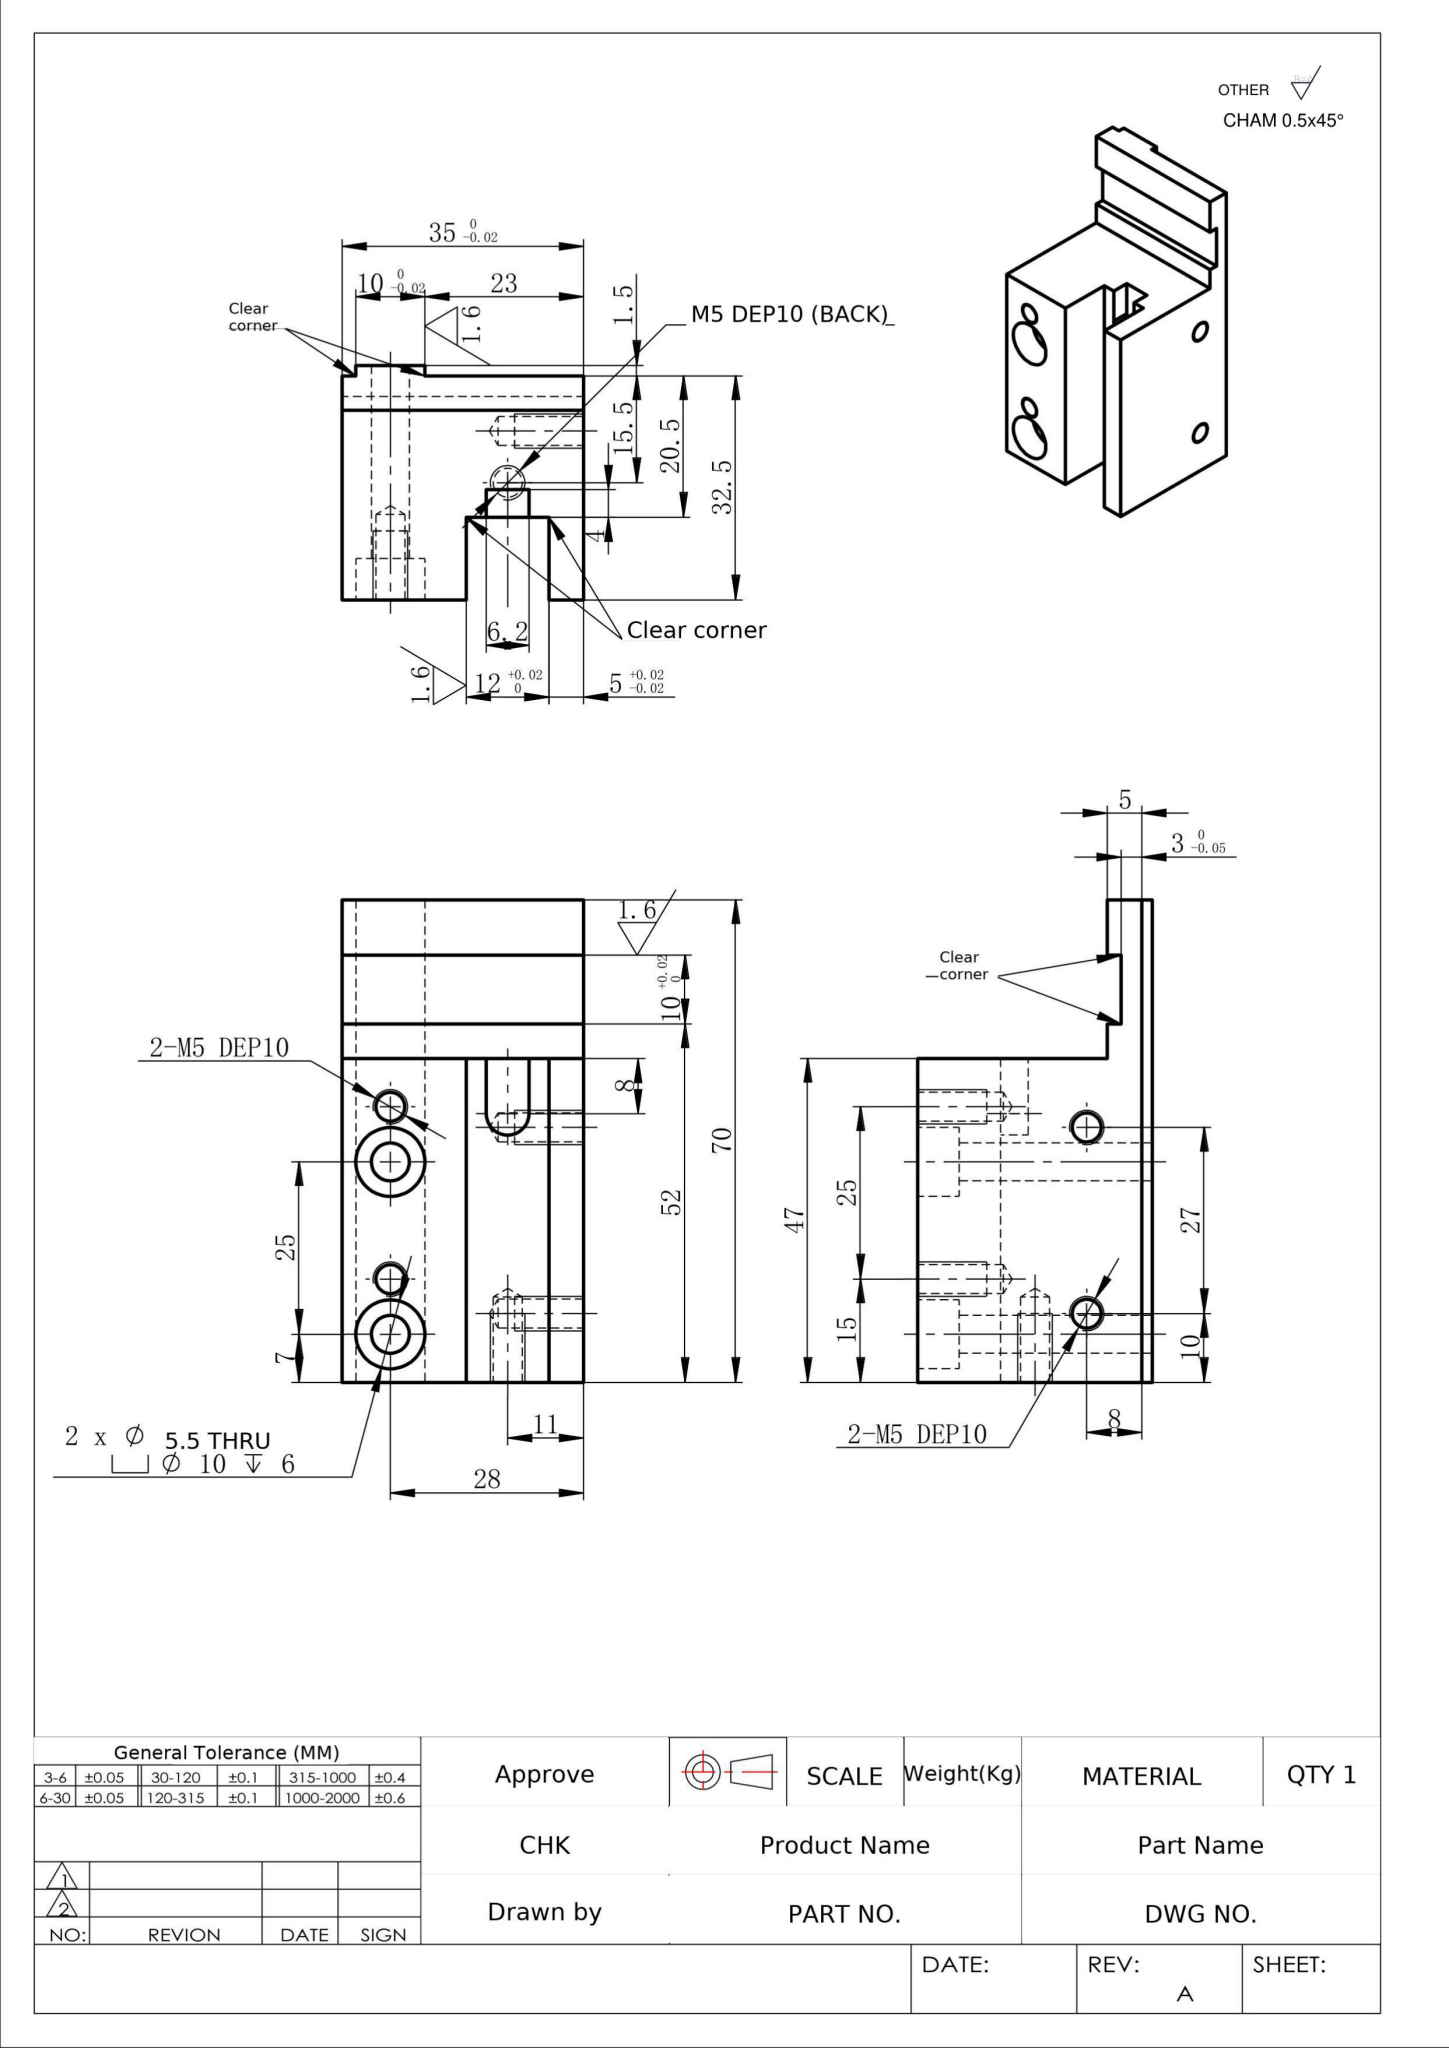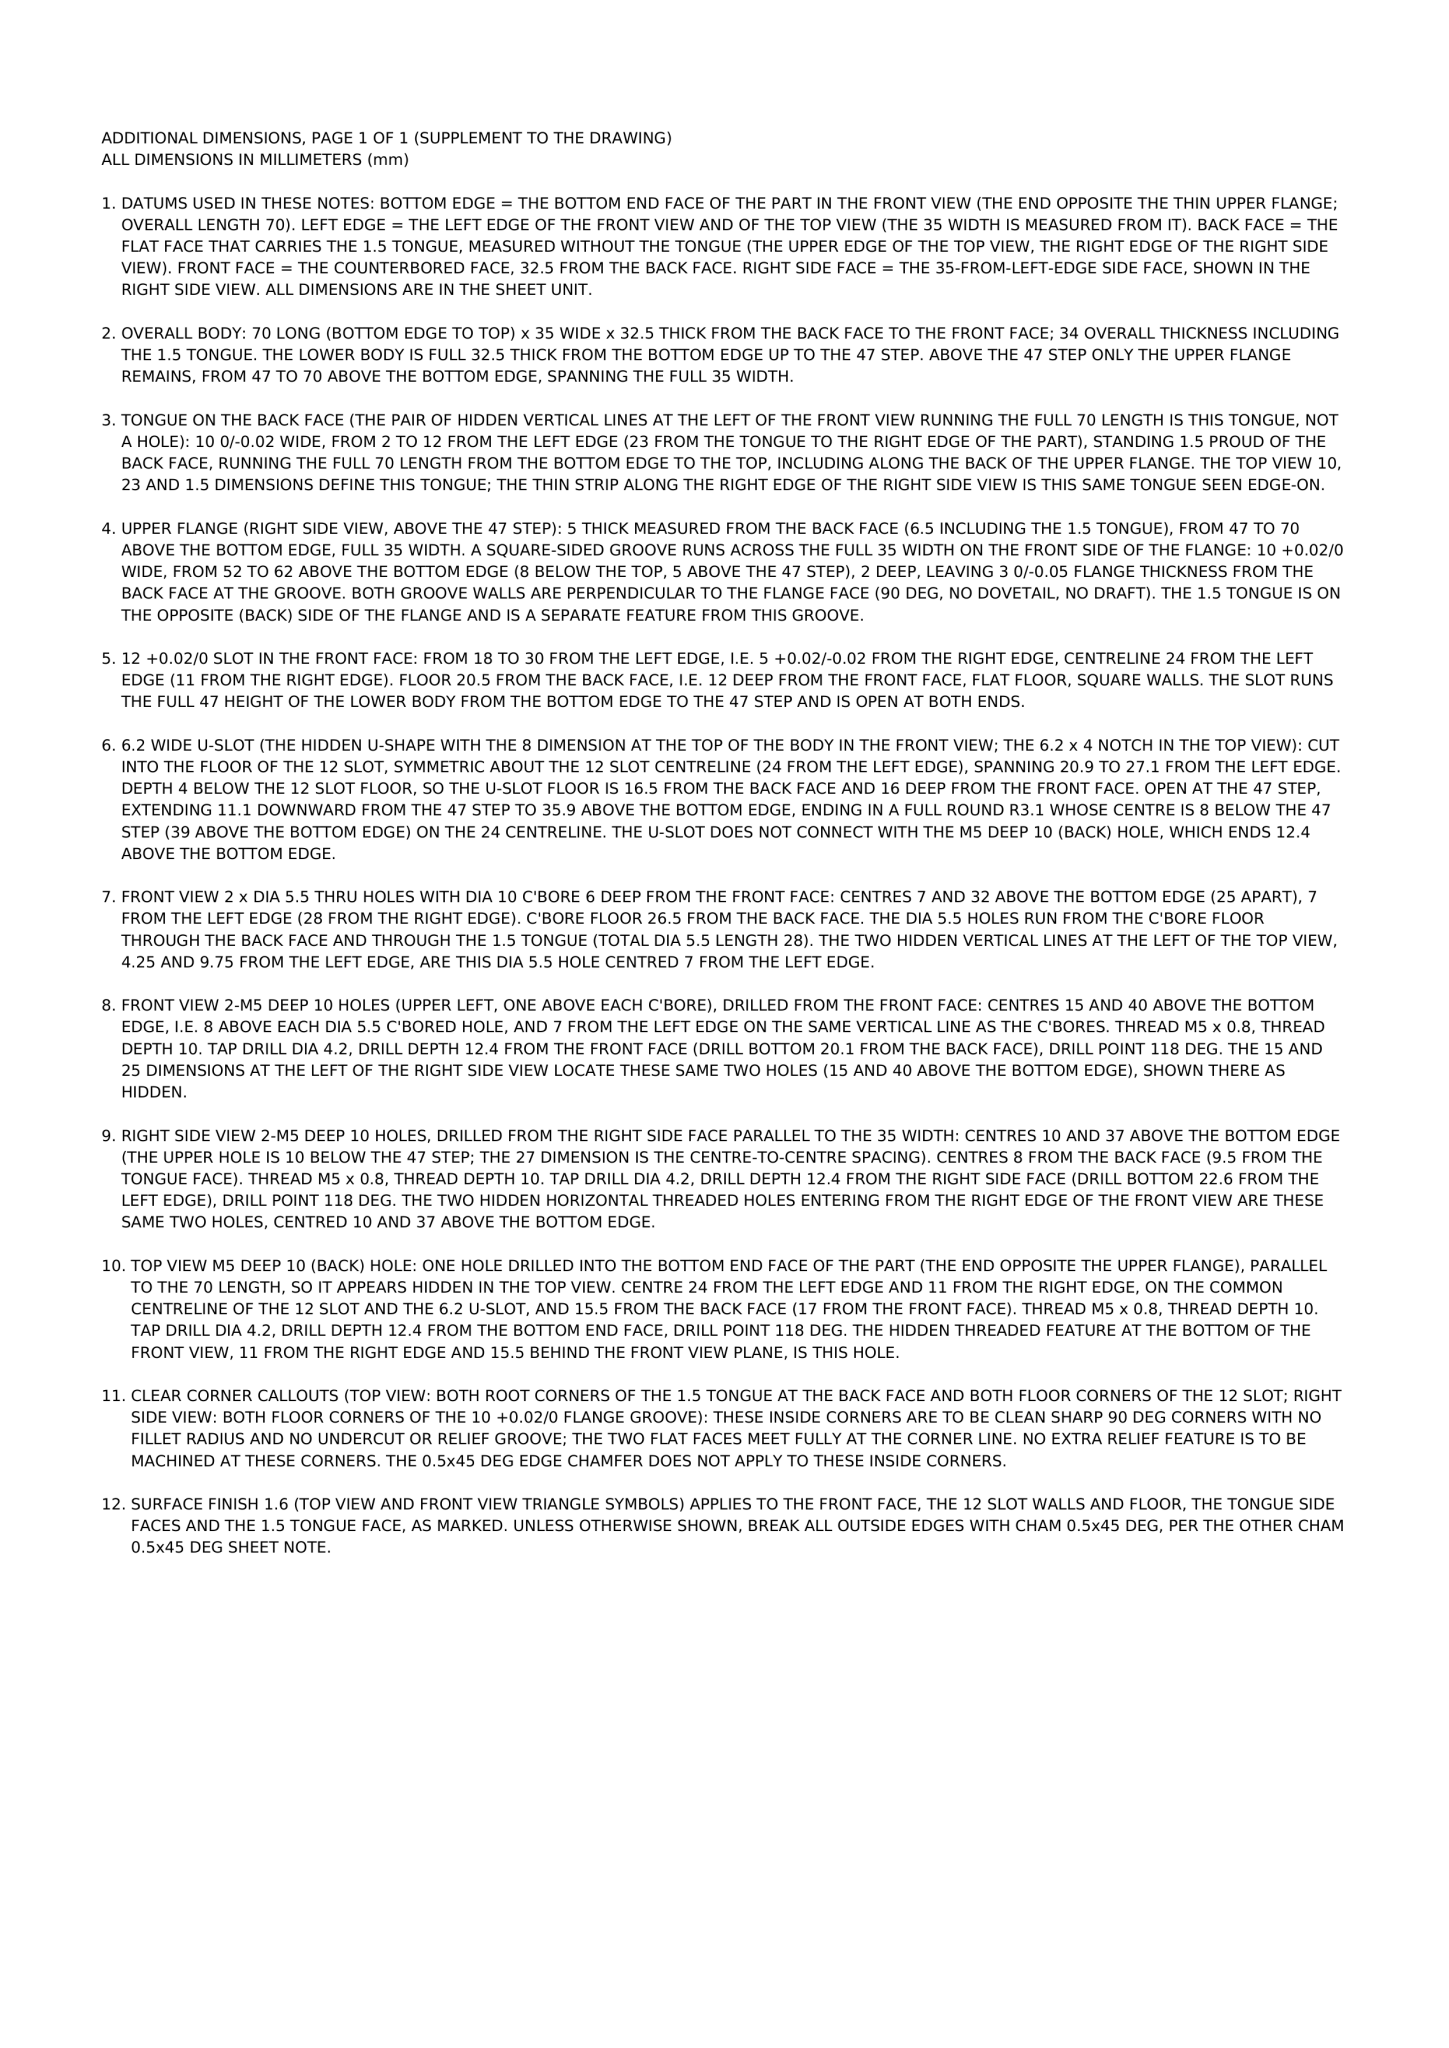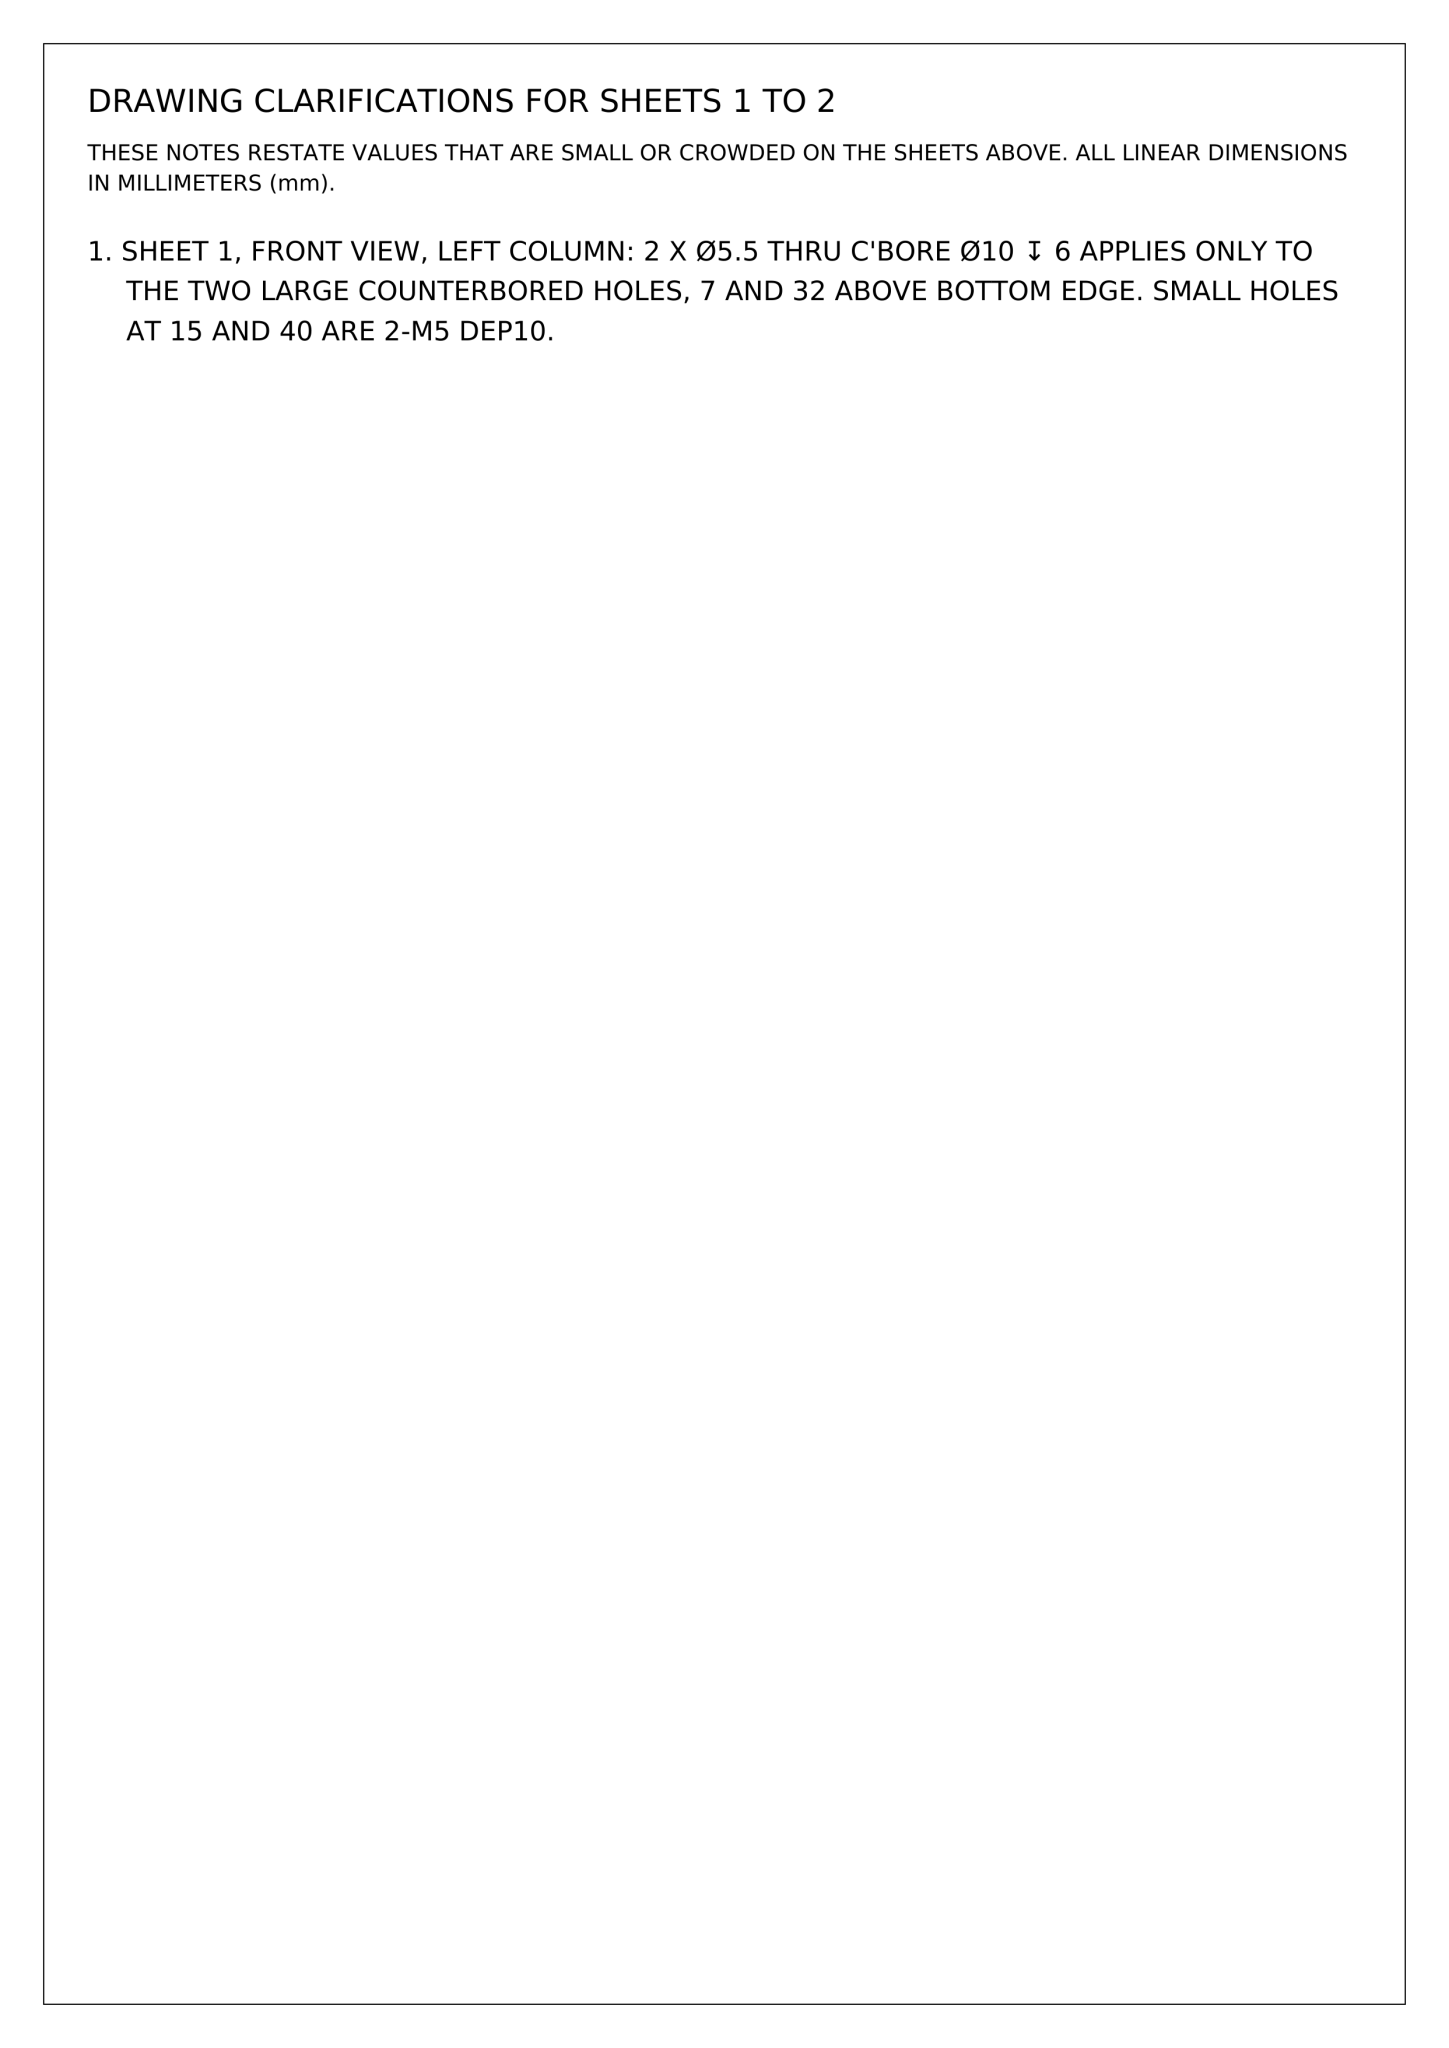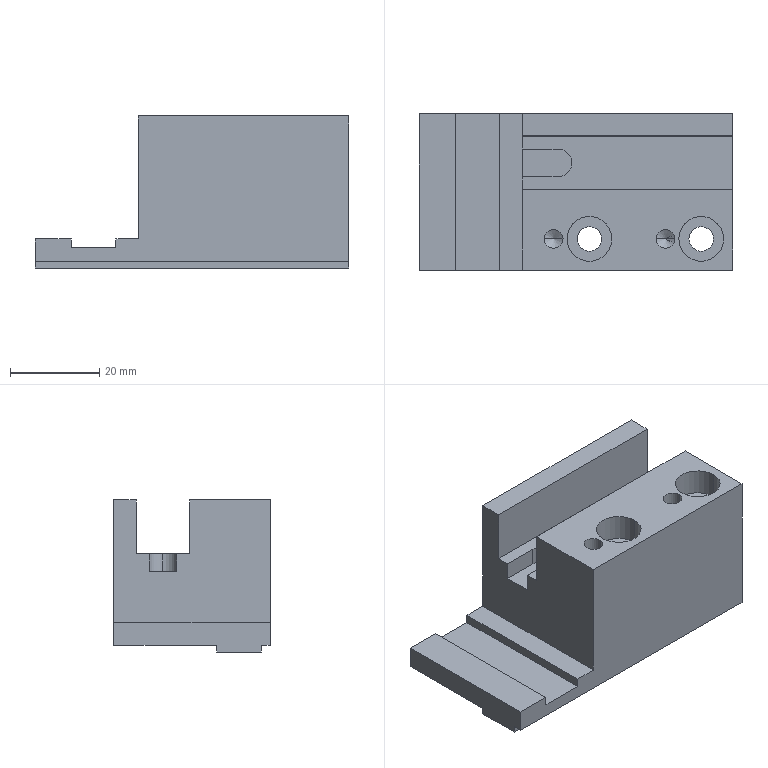Part | NX | mm | 1 solid | 55 faces | box 70 x 35 x 34 mm | volume 47650 mm3 | plane 25 | cylinder 20 | cone 10 | commonest cylinder face diameters 4.2 x10 10 x4 5.5 x4 6.2 x2